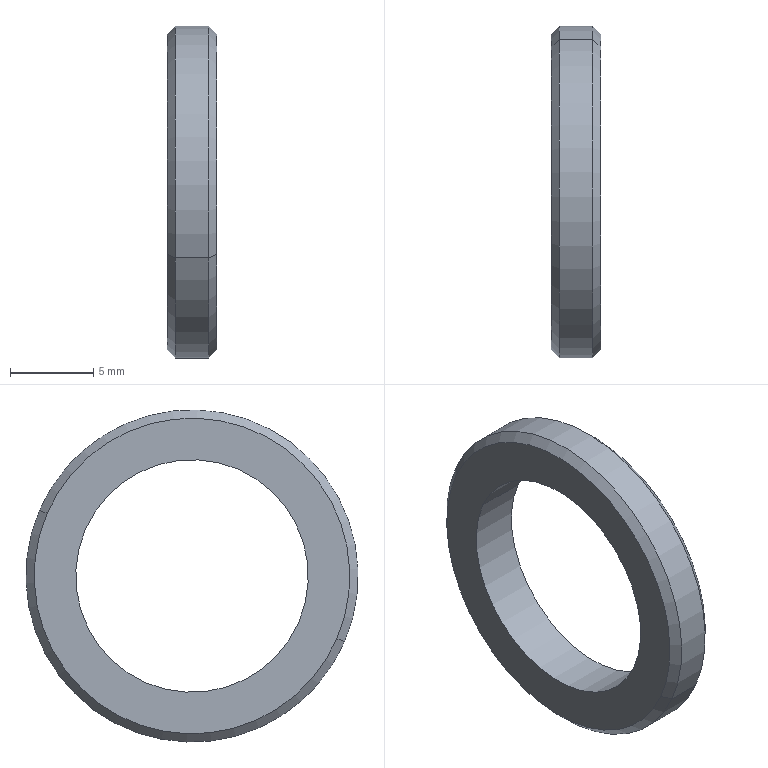Component | SolidWorks | 14Washer-1 | 1 solid | 10 faces | box 3 x 20 x 20 mm | volume 465 mm3 | cone 4 | cylinder 4 | plane 2 | commonest cylinder face diameters 14 x2 20 x2
build123d program:
from build123d import *

# Parameters (mm, degrees)
SKETCH1_R           = 10
SKETCH1_R_2         = 7
BOSS_EXTRUDE1_DEPTH = 3
CHAMFER1_SIZE       = 0.5


with BuildPart() as part:
    # Sketch1 → Boss-Extrude1 (new body)
    with BuildSketch(Plane.XY):
        Circle(SKETCH1_R)
        Circle(SKETCH1_R_2, mode=Mode.SUBTRACT)
    extrude(amount=BOSS_EXTRUDE1_DEPTH)

    # Chamfer1
    chamfer1_edges = [part.edges().sort_by_distance(p)[0] for p in [
        (-10, 0, 0),
        (-10, 0, 3),
    ]]
    chamfer(chamfer1_edges, length=CHAMFER1_SIZE)


solid = part.part

# Placed as in the assembly
solid = solid.moved(Location((-219, 57, -113), (0, 90, 0)))
STEP:
#1=COLOUR_RGB('',0.7922,0.8196,0.9333);
#2=FILL_AREA_STYLE_COLOUR('',#1);
#3=FILL_AREA_STYLE('',(#2));
#4=SURFACE_STYLE_FILL_AREA(#3);
#5=SURFACE_SIDE_STYLE('',(#4));
#6=SURFACE_STYLE_USAGE(.BOTH.,#5);
#7=PRESENTATION_STYLE_ASSIGNMENT((#6));
#8=CARTESIAN_POINT('',(-8.622,2.587,-4.301));
#9=VERTEX_POINT('',#8);
#10=CARTESIAN_POINT('',(-8.622,1.901,-4.597));
#11=VERTEX_POINT('',#10);
#12=CARTESIAN_POINT('',(-8.622,2.244,-4.449));
#13=DIRECTION('',(-1.,-0.,0.));
#14=DIRECTION('',(0.,0.9181,0.3964));
#15=AXIS2_PLACEMENT_3D('',#12,#13,#14);
#16=CIRCLE('',#15,0.374);
#17=EDGE_CURVE('',#9,#11,#16,.T.);
#18=ORIENTED_EDGE('',*,*,#17,.F.);
#19=CARTESIAN_POINT('',(-8.602,2.606,-4.293));
#20=VERTEX_POINT('',#19);
#21=CARTESIAN_POINT('',(-8.622,2.587,-4.301));
#22=DIRECTION('',(0.7071,0.6492,0.2803));
#23=VECTOR('',#22,39.37);
#24=LINE('',#21,#23);
#25=EDGE_CURVE('',#9,#20,#24,.T.);
#26=ORIENTED_EDGE('',*,*,#25,.T.);
#27=CARTESIAN_POINT('',(-8.602,1.883,-4.605));
#28=VERTEX_POINT('',#27);
#29=CARTESIAN_POINT('',(-8.602,2.244,-4.449));
#30=DIRECTION('',(1.,0.,-0.));
#31=DIRECTION('',(0.,0.9181,0.3964));
#32=AXIS2_PLACEMENT_3D('',#29,#30,#31);
#33=CIRCLE('',#32,0.3937);
#34=EDGE_CURVE('',#28,#20,#33,.T.);
#35=ORIENTED_EDGE('',*,*,#34,.F.);
#36=CARTESIAN_POINT('',(-8.622,1.901,-4.597));
#37=DIRECTION('',(0.7071,-0.6492,-0.2803));
#38=VECTOR('',#37,39.37);
#39=LINE('',#36,#38);
#40=EDGE_CURVE('',#11,#28,#39,.T.);
#41=ORIENTED_EDGE('',*,*,#40,.F.);
#42=EDGE_LOOP('',(#18,#26,#35,#41));
#43=FACE_OUTER_BOUND('',#42,.T.);
#44=CARTESIAN_POINT('',(-8.622,2.244,-4.449));
#45=DIRECTION('',(1.,0.,-0.));
#46=DIRECTION('',(0.,-0.9181,-0.3964));
#47=AXIS2_PLACEMENT_3D('',#44,#45,#46);
#48=CONICAL_SURFACE('',#47,0.374,0.7854);
#49=ADVANCED_FACE('',(#43),#48,.T.);
#50=CARTESIAN_POINT('',(-8.504,1.901,-4.597));
#51=VERTEX_POINT('',#50);
#52=CARTESIAN_POINT('',(-8.504,2.587,-4.301));
#53=VERTEX_POINT('',#52);
#54=CARTESIAN_POINT('',(-8.504,2.244,-4.449));
#55=DIRECTION('',(1.,0.,-0.));
#56=DIRECTION('',(0.,0.9181,0.3964));
#57=AXIS2_PLACEMENT_3D('',#54,#55,#56);
#58=CIRCLE('',#57,0.374);
#59=EDGE_CURVE('',#51,#53,#58,.T.);
#60=ORIENTED_EDGE('',*,*,#59,.F.);
#61=CARTESIAN_POINT('',(-8.524,1.883,-4.605));
#62=VERTEX_POINT('',#61);
#63=CARTESIAN_POINT('',(-8.524,1.883,-4.605));
#64=DIRECTION('',(-0.7071,-0.6492,-0.2803));
#65=VECTOR('',#64,39.37);
#66=LINE('',#63,#65);
#67=EDGE_CURVE('',#51,#62,#66,.T.);
#68=ORIENTED_EDGE('',*,*,#67,.T.);
#69=CARTESIAN_POINT('',(-8.524,2.606,-4.293));
#70=VERTEX_POINT('',#69);
#71=CARTESIAN_POINT('',(-8.524,2.244,-4.449));
#72=DIRECTION('',(-1.,-0.,0.));
#73=DIRECTION('',(0.,0.9181,0.3964));
#74=AXIS2_PLACEMENT_3D('',#71,#72,#73);
#75=CIRCLE('',#74,0.3937);
#76=EDGE_CURVE('',#70,#62,#75,.T.);
#77=ORIENTED_EDGE('',*,*,#76,.F.);
#78=CARTESIAN_POINT('',(-8.524,2.606,-4.293));
#79=DIRECTION('',(-0.7071,0.6492,0.2803));
#80=VECTOR('',#79,39.37);
#81=LINE('',#78,#80);
#82=EDGE_CURVE('',#53,#70,#81,.T.);
#83=ORIENTED_EDGE('',*,*,#82,.F.);
#84=EDGE_LOOP('',(#60,#68,#77,#83));
#85=FACE_OUTER_BOUND('',#84,.T.);
#86=CARTESIAN_POINT('',(-8.524,2.244,-4.449));
#87=DIRECTION('',(-1.,-0.,0.));
#88=DIRECTION('',(0.,0.9181,0.3964));
#89=AXIS2_PLACEMENT_3D('',#86,#87,#88);
#90=CONICAL_SURFACE('',#89,0.3937,0.7854);
#91=ADVANCED_FACE('',(#85),#90,.T.);
#92=CARTESIAN_POINT('',(-8.622,1.991,-4.558));
#93=VERTEX_POINT('',#92);
#94=CARTESIAN_POINT('',(-8.622,2.497,-4.34));
#95=VERTEX_POINT('',#94);
#96=CARTESIAN_POINT('',(-8.622,2.244,-4.449));
#97=DIRECTION('',(-1.,-0.,0.));
#98=DIRECTION('',(0.,0.9181,0.3964));
#99=AXIS2_PLACEMENT_3D('',#96,#97,#98);
#100=CIRCLE('',#99,0.2756);
#101=EDGE_CURVE('',#93,#95,#100,.T.);
#102=ORIENTED_EDGE('',*,*,#101,.T.);
#103=CARTESIAN_POINT('',(-8.504,2.497,-4.34));
#104=VERTEX_POINT('',#103);
#105=CARTESIAN_POINT('',(-8.622,2.497,-4.34));
#106=DIRECTION('',(1.,0.,-0.));
#107=VECTOR('',#106,39.37);
#108=LINE('',#105,#107);
#109=EDGE_CURVE('',#95,#104,#108,.T.);
#110=ORIENTED_EDGE('',*,*,#109,.T.);
#111=CARTESIAN_POINT('',(-8.504,1.991,-4.558));
#112=VERTEX_POINT('',#111);
#113=CARTESIAN_POINT('',(-8.504,2.244,-4.449));
#114=DIRECTION('',(-1.,-0.,0.));
#115=DIRECTION('',(0.,0.9181,0.3964));
#116=AXIS2_PLACEMENT_3D('',#113,#114,#115);
#117=CIRCLE('',#116,0.2756);
#118=EDGE_CURVE('',#112,#104,#117,.T.);
#119=ORIENTED_EDGE('',*,*,#118,.F.);
#120=CARTESIAN_POINT('',(-8.622,1.991,-4.558));
#121=DIRECTION('',(1.,0.,-0.));
#122=VECTOR('',#121,39.37);
#123=LINE('',#120,#122);
#124=EDGE_CURVE('',#93,#112,#123,.T.);
#125=ORIENTED_EDGE('',*,*,#124,.F.);
#126=EDGE_LOOP('',(#102,#110,#119,#125));
#127=FACE_OUTER_BOUND('',#126,.T.);
#128=CARTESIAN_POINT('',(-8.622,2.244,-4.449));
#129=DIRECTION('',(1.,0.,-0.));
#130=DIRECTION('',(0.,-0.9181,-0.3964));
#131=AXIS2_PLACEMENT_3D('',#128,#129,#130);
#132=CYLINDRICAL_SURFACE('',#131,0.2756);
#133=ADVANCED_FACE('',(#127),#132,.F.);
#134=ORIENTED_EDGE('',*,*,#34,.T.);
#135=CARTESIAN_POINT('',(-8.622,2.606,-4.293));
#136=DIRECTION('',(1.,0.,-0.));
#137=VECTOR('',#136,39.37);
#138=LINE('',#135,#137);
#139=EDGE_CURVE('',#20,#70,#138,.T.);
#140=ORIENTED_EDGE('',*,*,#139,.T.);
#141=ORIENTED_EDGE('',*,*,#76,.T.);
#142=CARTESIAN_POINT('',(-8.622,1.883,-4.605));
#143=DIRECTION('',(1.,0.,-0.));
#144=VECTOR('',#143,39.37);
#145=LINE('',#142,#144);
#146=EDGE_CURVE('',#28,#62,#145,.T.);
#147=ORIENTED_EDGE('',*,*,#146,.F.);
#148=EDGE_LOOP('',(#134,#140,#141,#147));
#149=FACE_OUTER_BOUND('',#148,.T.);
#150=CARTESIAN_POINT('',(-8.622,2.244,-4.449));
#151=DIRECTION('',(1.,0.,-0.));
#152=DIRECTION('',(0.,-0.9181,-0.3964));
#153=AXIS2_PLACEMENT_3D('',#150,#151,#152);
#154=CYLINDRICAL_SURFACE('',#153,0.3937);
#155=ADVANCED_FACE('',(#149),#154,.T.);
#156=CARTESIAN_POINT('',(-8.622,2.244,-4.449));
#157=DIRECTION('',(-1.,-0.,0.));
#158=DIRECTION('',(0.,0.9181,0.3964));
#159=AXIS2_PLACEMENT_3D('',#156,#157,#158);
#160=CIRCLE('',#159,0.374);
#161=EDGE_CURVE('',#11,#9,#160,.T.);
#162=ORIENTED_EDGE('',*,*,#161,.T.);
#163=ORIENTED_EDGE('',*,*,#17,.T.);
#164=EDGE_LOOP('',(#162,#163));
#165=FACE_OUTER_BOUND('',#164,.T.);
#166=ORIENTED_EDGE('',*,*,#101,.F.);
#167=CARTESIAN_POINT('',(-8.622,2.244,-4.449));
#168=DIRECTION('',(-1.,-0.,0.));
#169=DIRECTION('',(0.,0.9181,0.3964));
#170=AXIS2_PLACEMENT_3D('',#167,#168,#169);
#171=CIRCLE('',#170,0.2756);
#172=EDGE_CURVE('',#95,#93,#171,.T.);
#173=ORIENTED_EDGE('',*,*,#172,.F.);
#174=EDGE_LOOP('',(#166,#173));
#175=FACE_BOUND('',#174,.T.);
#176=CARTESIAN_POINT('',(-8.622,2.244,-4.449));
#177=DIRECTION('',(-1.,-0.,0.));
#178=DIRECTION('',(0.,0.9181,0.3964));
#179=AXIS2_PLACEMENT_3D('',#176,#177,#178);
#180=PLANE('',#179);
#181=ADVANCED_FACE('',(#165,#175),#180,.T.);
#182=CARTESIAN_POINT('',(-8.504,2.244,-4.449));
#183=DIRECTION('',(1.,0.,-0.));
#184=DIRECTION('',(0.,0.9181,0.3964));
#185=AXIS2_PLACEMENT_3D('',#182,#183,#184);
#186=CIRCLE('',#185,0.374);
#187=EDGE_CURVE('',#53,#51,#186,.T.);
#188=ORIENTED_EDGE('',*,*,#187,.T.);
#189=ORIENTED_EDGE('',*,*,#59,.T.);
#190=EDGE_LOOP('',(#188,#189));
#191=FACE_OUTER_BOUND('',#190,.T.);
#192=ORIENTED_EDGE('',*,*,#118,.T.);
#193=CARTESIAN_POINT('',(-8.504,2.244,-4.449));
#194=DIRECTION('',(-1.,-0.,0.));
#195=DIRECTION('',(0.,0.9181,0.3964));
#196=AXIS2_PLACEMENT_3D('',#193,#194,#195);
#197=CIRCLE('',#196,0.2756);
#198=EDGE_CURVE('',#104,#112,#197,.T.);
#199=ORIENTED_EDGE('',*,*,#198,.T.);
#200=EDGE_LOOP('',(#192,#199));
#201=FACE_BOUND('',#200,.T.);
#202=CARTESIAN_POINT('',(-8.504,2.244,-4.449));
#203=DIRECTION('',(-1.,-0.,0.));
#204=DIRECTION('',(0.,0.9181,0.3964));
#205=AXIS2_PLACEMENT_3D('',#202,#203,#204);
#206=PLANE('',#205);
#207=ADVANCED_FACE('',(#191,#201),#206,.F.);
#208=ORIENTED_EDGE('',*,*,#139,.F.);
#209=CARTESIAN_POINT('',(-8.602,2.244,-4.449));
#210=DIRECTION('',(1.,0.,-0.));
#211=DIRECTION('',(0.,0.9181,0.3964));
#212=AXIS2_PLACEMENT_3D('',#209,#210,#211);
#213=CIRCLE('',#212,0.3937);
#214=EDGE_CURVE('',#20,#28,#213,.T.);
#215=ORIENTED_EDGE('',*,*,#214,.T.);
#216=ORIENTED_EDGE('',*,*,#146,.T.);
#217=CARTESIAN_POINT('',(-8.524,2.244,-4.449));
#218=DIRECTION('',(-1.,-0.,0.));
#219=DIRECTION('',(0.,0.9181,0.3964));
#220=AXIS2_PLACEMENT_3D('',#217,#218,#219);
#221=CIRCLE('',#220,0.3937);
#222=EDGE_CURVE('',#62,#70,#221,.T.);
#223=ORIENTED_EDGE('',*,*,#222,.T.);
#224=EDGE_LOOP('',(#208,#215,#216,#223));
#225=FACE_OUTER_BOUND('',#224,.T.);
#226=CARTESIAN_POINT('',(-8.622,2.244,-4.449));
#227=DIRECTION('',(1.,0.,-0.));
#228=DIRECTION('',(0.,-0.9181,-0.3964));
#229=AXIS2_PLACEMENT_3D('',#226,#227,#228);
#230=CYLINDRICAL_SURFACE('',#229,0.3937);
#231=ADVANCED_FACE('',(#225),#230,.T.);
#232=ORIENTED_EDGE('',*,*,#109,.F.);
#233=ORIENTED_EDGE('',*,*,#172,.T.);
#234=ORIENTED_EDGE('',*,*,#124,.T.);
#235=ORIENTED_EDGE('',*,*,#198,.F.);
#236=EDGE_LOOP('',(#232,#233,#234,#235));
#237=FACE_OUTER_BOUND('',#236,.T.);
#238=CARTESIAN_POINT('',(-8.622,2.244,-4.449));
#239=DIRECTION('',(1.,0.,-0.));
#240=DIRECTION('',(0.,-0.9181,-0.3964));
#241=AXIS2_PLACEMENT_3D('',#238,#239,#240);
#242=CYLINDRICAL_SURFACE('',#241,0.2756);
#243=ADVANCED_FACE('',(#237),#242,.F.);
#244=ORIENTED_EDGE('',*,*,#67,.F.);
#245=ORIENTED_EDGE('',*,*,#187,.F.);
#246=ORIENTED_EDGE('',*,*,#82,.T.);
#247=ORIENTED_EDGE('',*,*,#222,.F.);
#248=EDGE_LOOP('',(#244,#245,#246,#247));
#249=FACE_OUTER_BOUND('',#248,.T.);
#250=CARTESIAN_POINT('',(-8.524,2.244,-4.449));
#251=DIRECTION('',(-1.,-0.,0.));
#252=DIRECTION('',(0.,0.9181,0.3964));
#253=AXIS2_PLACEMENT_3D('',#250,#251,#252);
#254=CONICAL_SURFACE('',#253,0.3937,0.7854);
#255=ADVANCED_FACE('',(#249),#254,.T.);
#256=ORIENTED_EDGE('',*,*,#25,.F.);
#257=ORIENTED_EDGE('',*,*,#161,.F.);
#258=ORIENTED_EDGE('',*,*,#40,.T.);
#259=ORIENTED_EDGE('',*,*,#214,.F.);
#260=EDGE_LOOP('',(#256,#257,#258,#259));
#261=FACE_OUTER_BOUND('',#260,.T.);
#262=CARTESIAN_POINT('',(-8.622,2.244,-4.449));
#263=DIRECTION('',(1.,0.,-0.));
#264=DIRECTION('',(0.,-0.9181,-0.3964));
#265=AXIS2_PLACEMENT_3D('',#262,#263,#264);
#266=CONICAL_SURFACE('',#265,0.374,0.7854);
#267=ADVANCED_FACE('',(#261),#266,.T.);
#268=CLOSED_SHELL('',(#49,#91,#133,#155,#181,#207,#231,#243,#255,#267));
#269=MANIFOLD_SOLID_BREP('',#268);
#270=STYLED_ITEM('',(#7),#269);
#271=PRESENTATION_LAYER_ASSIGNMENT('','',(#270));
#272=(LENGTH_UNIT()NAMED_UNIT(*)SI_UNIT($,.METRE.));
#273=LENGTH_MEASURE_WITH_UNIT(LENGTH_MEASURE(0.0254),#272);
#274=DIMENSIONAL_EXPONENTS(1.,0.,0.,0.,0.,0.,0.);
#275=(CONVERSION_BASED_UNIT('',#273)LENGTH_UNIT()NAMED_UNIT(#274));
#276=UNCERTAINTY_MEASURE_WITH_UNIT(LENGTH_MEASURE(0.00001),#275,'','');
#277=(NAMED_UNIT(*)PLANE_ANGLE_UNIT()SI_UNIT($,.RADIAN.));
#278=(NAMED_UNIT(*)SI_UNIT($,.STERADIAN.)SOLID_ANGLE_UNIT());
#279=(GEOMETRIC_REPRESENTATION_CONTEXT(3)GLOBAL_UNCERTAINTY_ASSIGNED_CONTEXT((#276))GLOBAL_UNIT_ASSIGNED_CONTEXT((#275,#277,#278))REPRESENTATION_CONTEXT('',''));
#280=MECHANICAL_DESIGN_GEOMETRIC_PRESENTATION_REPRESENTATION('',(#270),#279);
#281=CARTESIAN_POINT('',(0.,0.,0.));
#282=DIRECTION('',(0.,0.,1.));
#283=DIRECTION('',(1.,0.,0.));
#284=AXIS2_PLACEMENT_3D('',#281,#282,#283);
#285=(LENGTH_UNIT()NAMED_UNIT(*)SI_UNIT($,.METRE.));
#286=LENGTH_MEASURE_WITH_UNIT(LENGTH_MEASURE(0.0254),#285);
#287=DIMENSIONAL_EXPONENTS(1.,0.,0.,0.,0.,0.,0.);
#288=(CONVERSION_BASED_UNIT('',#286)LENGTH_UNIT()NAMED_UNIT(#287));
#289=UNCERTAINTY_MEASURE_WITH_UNIT(LENGTH_MEASURE(0.00001),#288,'','');
#290=(NAMED_UNIT(*)PLANE_ANGLE_UNIT()SI_UNIT($,.RADIAN.));
#291=(NAMED_UNIT(*)SI_UNIT($,.STERADIAN.)SOLID_ANGLE_UNIT());
#292=(GEOMETRIC_REPRESENTATION_CONTEXT(3)GLOBAL_UNCERTAINTY_ASSIGNED_CONTEXT((#289))GLOBAL_UNIT_ASSIGNED_CONTEXT((#288,#290,#291))REPRESENTATION_CONTEXT('',''));
#293=ADVANCED_BREP_SHAPE_REPRESENTATION('',(#269,#284),#292);